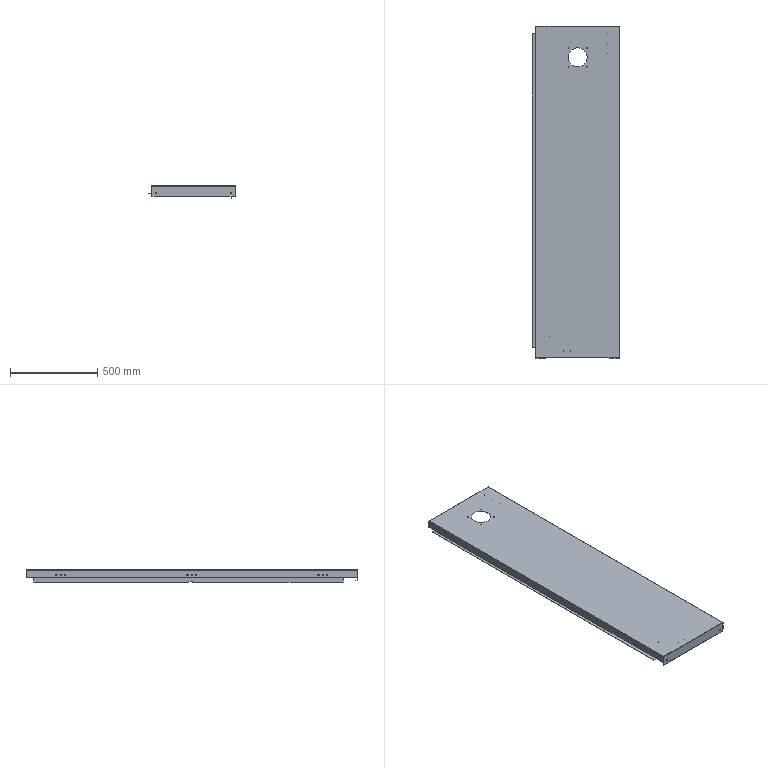Component | SolidWorks | CabinetWelding-1_RightSidePlate-1 | 1 solid | 140 faces | volume 1452182 mm3 | cylinder 80 | plane 50 | spline 10 | commonest cylinder face diameters 4 x22 7 x18 0.5 x12 5 x8 0.2 x7 2.6 x7 8.5 x4 110 x2